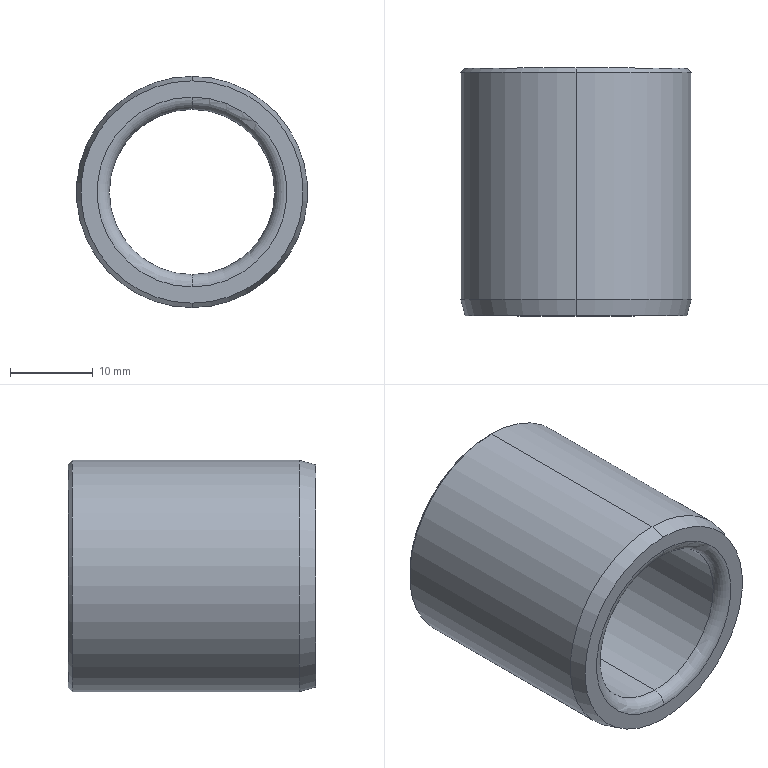Component | SolidWorks | BearingLiftingModule-1_CylinderLiftingModule-1_OFG01-d20-L30-1 | 1 solid | 14 faces | box 28 x 30 x 28 mm | volume 8928 mm3 | cone 4 | torus 4 | cylinder 4 | plane 2 | commonest cylinder face diameters 20 x2 28 x2
STEP:
#1=COLOUR_RGB('',0.7922,0.8196,0.9333);
#2=FILL_AREA_STYLE_COLOUR('',#1);
#3=FILL_AREA_STYLE('',(#2));
#4=SURFACE_STYLE_FILL_AREA(#3);
#5=SURFACE_SIDE_STYLE('',(#4));
#6=SURFACE_STYLE_USAGE(.BOTH.,#5);
#7=PRESENTATION_STYLE_ASSIGNMENT((#6));
#8=CARTESIAN_POINT('',(2.756,-1.622,1.711));
#9=VERTEX_POINT('',#8);
#10=CARTESIAN_POINT('',(2.756,-1.622,0.651));
#11=VERTEX_POINT('',#10);
#12=CARTESIAN_POINT('',(2.756,-1.622,1.181));
#13=DIRECTION('',(0.,-1.,0.));
#14=DIRECTION('',(0.,0.,1.));
#15=AXIS2_PLACEMENT_3D('',#12,#13,#14);
#16=CIRCLE('',#15,0.5301);
#17=EDGE_CURVE('',#9,#11,#16,.T.);
#18=ORIENTED_EDGE('',*,*,#17,.F.);
#19=CARTESIAN_POINT('',(2.756,-1.543,1.732));
#20=VERTEX_POINT('',#19);
#21=CARTESIAN_POINT('',(2.756,-1.622,1.711));
#22=DIRECTION('',(-0.,0.9659,0.2588));
#23=VECTOR('',#22,39.37);
#24=LINE('',#21,#23);
#25=EDGE_CURVE('',#9,#20,#24,.T.);
#26=ORIENTED_EDGE('',*,*,#25,.T.);
#27=CARTESIAN_POINT('',(2.756,-1.543,0.6299));
#28=VERTEX_POINT('',#27);
#29=CARTESIAN_POINT('',(2.756,-1.543,1.181));
#30=DIRECTION('',(0.,-1.,0.));
#31=DIRECTION('',(0.,0.,1.));
#32=AXIS2_PLACEMENT_3D('',#29,#30,#31);
#33=CIRCLE('',#32,0.5512);
#34=EDGE_CURVE('',#20,#28,#33,.T.);
#35=ORIENTED_EDGE('',*,*,#34,.T.);
#36=CARTESIAN_POINT('',(2.756,-1.622,0.651));
#37=DIRECTION('',(-0.,0.9659,-0.2588));
#38=VECTOR('',#37,39.37);
#39=LINE('',#36,#38);
#40=EDGE_CURVE('',#11,#28,#39,.T.);
#41=ORIENTED_EDGE('',*,*,#40,.F.);
#42=EDGE_LOOP('',(#18,#26,#35,#41));
#43=FACE_OUTER_BOUND('',#42,.T.);
#44=CARTESIAN_POINT('',(2.756,-1.622,1.181));
#45=DIRECTION('',(0.,1.,-0.));
#46=DIRECTION('',(0.,0.,-1.));
#47=AXIS2_PLACEMENT_3D('',#44,#45,#46);
#48=CONICAL_SURFACE('',#47,0.5301,0.2618);
#49=ADVANCED_FACE('',(#43),#48,.T.);
#50=CARTESIAN_POINT('',(2.756,-1.622,1.634));
#51=VERTEX_POINT('',#50);
#52=CARTESIAN_POINT('',(2.756,-1.622,0.7283));
#53=VERTEX_POINT('',#52);
#54=CARTESIAN_POINT('',(2.756,-1.622,1.181));
#55=DIRECTION('',(0.,-1.,0.));
#56=DIRECTION('',(0.,0.,1.));
#57=AXIS2_PLACEMENT_3D('',#54,#55,#56);
#58=CIRCLE('',#57,0.4528);
#59=EDGE_CURVE('',#51,#53,#58,.T.);
#60=ORIENTED_EDGE('',*,*,#59,.T.);
#61=CARTESIAN_POINT('',(2.756,-1.563,0.7874));
#62=VERTEX_POINT('',#61);
#63=CARTESIAN_POINT('',(2.756,-1.563,0.7283));
#64=DIRECTION('',(-1.,0.,0.));
#65=DIRECTION('',(0.,0.,1.));
#66=AXIS2_PLACEMENT_3D('',#63,#64,#65);
#67=CIRCLE('',#66,0.05906);
#68=EDGE_CURVE('',#53,#62,#67,.T.);
#69=ORIENTED_EDGE('',*,*,#68,.T.);
#70=CARTESIAN_POINT('',(2.756,-1.563,1.575));
#71=VERTEX_POINT('',#70);
#72=CARTESIAN_POINT('',(2.756,-1.563,1.181));
#73=DIRECTION('',(0.,-1.,0.));
#74=DIRECTION('',(0.,0.,1.));
#75=AXIS2_PLACEMENT_3D('',#72,#73,#74);
#76=CIRCLE('',#75,0.3937);
#77=EDGE_CURVE('',#71,#62,#76,.T.);
#78=ORIENTED_EDGE('',*,*,#77,.F.);
#79=CARTESIAN_POINT('',(2.756,-1.563,1.634));
#80=DIRECTION('',(1.,-0.,-0.));
#81=DIRECTION('',(0.,0.,-1.));
#82=AXIS2_PLACEMENT_3D('',#79,#80,#81);
#83=CIRCLE('',#82,0.05906);
#84=EDGE_CURVE('',#51,#71,#83,.T.);
#85=ORIENTED_EDGE('',*,*,#84,.F.);
#86=EDGE_LOOP('',(#60,#69,#78,#85));
#87=FACE_OUTER_BOUND('',#86,.T.);
#88=CARTESIAN_POINT('',(2.756,-1.563,1.181));
#89=DIRECTION('',(0.,-1.,0.));
#90=DIRECTION('',(0.,0.,1.));
#91=AXIS2_PLACEMENT_3D('',#88,#89,#90);
#92=TOROIDAL_SURFACE('',#91,0.4528,0.05906);
#93=ADVANCED_FACE('',(#87),#92,.T.);
#94=ORIENTED_EDGE('',*,*,#77,.T.);
#95=CARTESIAN_POINT('',(2.756,-0.5,0.7874));
#96=VERTEX_POINT('',#95);
#97=CARTESIAN_POINT('',(2.756,-1.622,0.7874));
#98=DIRECTION('',(0.,1.,-0.));
#99=VECTOR('',#98,39.37);
#100=LINE('',#97,#99);
#101=EDGE_CURVE('',#62,#96,#100,.T.);
#102=ORIENTED_EDGE('',*,*,#101,.T.);
#103=CARTESIAN_POINT('',(2.756,-0.5,1.575));
#104=VERTEX_POINT('',#103);
#105=CARTESIAN_POINT('',(2.756,-0.5,1.181));
#106=DIRECTION('',(0.,-1.,0.));
#107=DIRECTION('',(0.,0.,1.));
#108=AXIS2_PLACEMENT_3D('',#105,#106,#107);
#109=CIRCLE('',#108,0.3937);
#110=EDGE_CURVE('',#104,#96,#109,.T.);
#111=ORIENTED_EDGE('',*,*,#110,.F.);
#112=CARTESIAN_POINT('',(2.756,-1.622,1.575));
#113=DIRECTION('',(0.,1.,-0.));
#114=VECTOR('',#113,39.37);
#115=LINE('',#112,#114);
#116=EDGE_CURVE('',#71,#104,#115,.T.);
#117=ORIENTED_EDGE('',*,*,#116,.F.);
#118=EDGE_LOOP('',(#94,#102,#111,#117));
#119=FACE_OUTER_BOUND('',#118,.T.);
#120=CARTESIAN_POINT('',(2.756,-1.622,1.181));
#121=DIRECTION('',(0.,1.,-0.));
#122=DIRECTION('',(0.,0.,1.));
#123=AXIS2_PLACEMENT_3D('',#120,#121,#122);
#124=CYLINDRICAL_SURFACE('',#123,0.3937);
#125=ADVANCED_FACE('',(#119),#124,.F.);
#126=ORIENTED_EDGE('',*,*,#110,.T.);
#127=CARTESIAN_POINT('',(2.756,-0.4409,0.7283));
#128=VERTEX_POINT('',#127);
#129=CARTESIAN_POINT('',(2.756,-0.5,0.7283));
#130=DIRECTION('',(-1.,0.,0.));
#131=DIRECTION('',(0.,0.,1.));
#132=AXIS2_PLACEMENT_3D('',#129,#130,#131);
#133=CIRCLE('',#132,0.05906);
#134=EDGE_CURVE('',#96,#128,#133,.T.);
#135=ORIENTED_EDGE('',*,*,#134,.T.);
#136=CARTESIAN_POINT('',(2.756,-0.4409,1.634));
#137=VERTEX_POINT('',#136);
#138=CARTESIAN_POINT('',(2.756,-0.4409,1.181));
#139=DIRECTION('',(0.,-1.,0.));
#140=DIRECTION('',(0.,0.,1.));
#141=AXIS2_PLACEMENT_3D('',#138,#139,#140);
#142=CIRCLE('',#141,0.4528);
#143=EDGE_CURVE('',#137,#128,#142,.T.);
#144=ORIENTED_EDGE('',*,*,#143,.F.);
#145=CARTESIAN_POINT('',(2.756,-0.5,1.634));
#146=DIRECTION('',(1.,-0.,-0.));
#147=DIRECTION('',(0.,0.,-1.));
#148=AXIS2_PLACEMENT_3D('',#145,#146,#147);
#149=CIRCLE('',#148,0.05906);
#150=EDGE_CURVE('',#104,#137,#149,.T.);
#151=ORIENTED_EDGE('',*,*,#150,.F.);
#152=EDGE_LOOP('',(#126,#135,#144,#151));
#153=FACE_OUTER_BOUND('',#152,.T.);
#154=CARTESIAN_POINT('',(2.756,-0.5,1.181));
#155=DIRECTION('',(0.,-1.,0.));
#156=DIRECTION('',(0.,0.,1.));
#157=AXIS2_PLACEMENT_3D('',#154,#155,#156);
#158=TOROIDAL_SURFACE('',#157,0.4528,0.05906);
#159=ADVANCED_FACE('',(#153),#158,.T.);
#160=CARTESIAN_POINT('',(2.756,-1.543,1.181));
#161=DIRECTION('',(0.,-1.,0.));
#162=DIRECTION('',(0.,0.,1.));
#163=AXIS2_PLACEMENT_3D('',#160,#161,#162);
#164=CIRCLE('',#163,0.5512);
#165=EDGE_CURVE('',#28,#20,#164,.T.);
#166=ORIENTED_EDGE('',*,*,#165,.F.);
#167=CARTESIAN_POINT('',(2.756,-0.4606,0.6299));
#168=VERTEX_POINT('',#167);
#169=CARTESIAN_POINT('',(2.756,-1.622,0.6299));
#170=DIRECTION('',(0.,1.,-0.));
#171=VECTOR('',#170,39.37);
#172=LINE('',#169,#171);
#173=EDGE_CURVE('',#28,#168,#172,.T.);
#174=ORIENTED_EDGE('',*,*,#173,.T.);
#175=CARTESIAN_POINT('',(2.756,-0.4606,1.732));
#176=VERTEX_POINT('',#175);
#177=CARTESIAN_POINT('',(2.756,-0.4606,1.181));
#178=DIRECTION('',(0.,-1.,0.));
#179=DIRECTION('',(0.,0.,1.));
#180=AXIS2_PLACEMENT_3D('',#177,#178,#179);
#181=CIRCLE('',#180,0.5512);
#182=EDGE_CURVE('',#168,#176,#181,.T.);
#183=ORIENTED_EDGE('',*,*,#182,.T.);
#184=CARTESIAN_POINT('',(2.756,-1.622,1.732));
#185=DIRECTION('',(0.,1.,-0.));
#186=VECTOR('',#185,39.37);
#187=LINE('',#184,#186);
#188=EDGE_CURVE('',#20,#176,#187,.T.);
#189=ORIENTED_EDGE('',*,*,#188,.F.);
#190=EDGE_LOOP('',(#166,#174,#183,#189));
#191=FACE_OUTER_BOUND('',#190,.T.);
#192=CARTESIAN_POINT('',(2.756,-1.622,1.181));
#193=DIRECTION('',(0.,1.,-0.));
#194=DIRECTION('',(0.,0.,1.));
#195=AXIS2_PLACEMENT_3D('',#192,#193,#194);
#196=CYLINDRICAL_SURFACE('',#195,0.5512);
#197=ADVANCED_FACE('',(#191),#196,.T.);
#198=CARTESIAN_POINT('',(2.756,-0.4409,1.713));
#199=VERTEX_POINT('',#198);
#200=CARTESIAN_POINT('',(2.756,-0.4409,0.6496));
#201=VERTEX_POINT('',#200);
#202=CARTESIAN_POINT('',(2.756,-0.4409,1.181));
#203=DIRECTION('',(0.,-1.,0.));
#204=DIRECTION('',(0.,0.,1.));
#205=AXIS2_PLACEMENT_3D('',#202,#203,#204);
#206=CIRCLE('',#205,0.5315);
#207=EDGE_CURVE('',#199,#201,#206,.T.);
#208=ORIENTED_EDGE('',*,*,#207,.T.);
#209=CARTESIAN_POINT('',(2.756,-0.4606,0.6299));
#210=DIRECTION('',(-0.,-0.7071,-0.7071));
#211=VECTOR('',#210,39.37);
#212=LINE('',#209,#211);
#213=EDGE_CURVE('',#201,#168,#212,.T.);
#214=ORIENTED_EDGE('',*,*,#213,.T.);
#215=CARTESIAN_POINT('',(2.756,-0.4606,1.181));
#216=DIRECTION('',(0.,-1.,0.));
#217=DIRECTION('',(0.,0.,1.));
#218=AXIS2_PLACEMENT_3D('',#215,#216,#217);
#219=CIRCLE('',#218,0.5512);
#220=EDGE_CURVE('',#176,#168,#219,.T.);
#221=ORIENTED_EDGE('',*,*,#220,.F.);
#222=CARTESIAN_POINT('',(2.756,-0.4606,1.732));
#223=DIRECTION('',(0.,-0.7071,0.7071));
#224=VECTOR('',#223,39.37);
#225=LINE('',#222,#224);
#226=EDGE_CURVE('',#199,#176,#225,.T.);
#227=ORIENTED_EDGE('',*,*,#226,.F.);
#228=EDGE_LOOP('',(#208,#214,#221,#227));
#229=FACE_OUTER_BOUND('',#228,.T.);
#230=CARTESIAN_POINT('',(2.756,-0.4606,1.181));
#231=DIRECTION('',(0.,-1.,0.));
#232=DIRECTION('',(0.,0.,1.));
#233=AXIS2_PLACEMENT_3D('',#230,#231,#232);
#234=CONICAL_SURFACE('',#233,0.5512,0.7854);
#235=ADVANCED_FACE('',(#229),#234,.T.);
#236=ORIENTED_EDGE('',*,*,#213,.F.);
#237=CARTESIAN_POINT('',(2.756,-0.4409,1.181));
#238=DIRECTION('',(0.,-1.,0.));
#239=DIRECTION('',(0.,0.,1.));
#240=AXIS2_PLACEMENT_3D('',#237,#238,#239);
#241=CIRCLE('',#240,0.5315);
#242=EDGE_CURVE('',#201,#199,#241,.T.);
#243=ORIENTED_EDGE('',*,*,#242,.T.);
#244=ORIENTED_EDGE('',*,*,#226,.T.);
#245=ORIENTED_EDGE('',*,*,#182,.F.);
#246=EDGE_LOOP('',(#236,#243,#244,#245));
#247=FACE_OUTER_BOUND('',#246,.T.);
#248=CARTESIAN_POINT('',(2.756,-0.4606,1.181));
#249=DIRECTION('',(0.,-1.,0.));
#250=DIRECTION('',(0.,0.,1.));
#251=AXIS2_PLACEMENT_3D('',#248,#249,#250);
#252=CONICAL_SURFACE('',#251,0.5512,0.7854);
#253=ADVANCED_FACE('',(#247),#252,.T.);
#254=ORIENTED_EDGE('',*,*,#173,.F.);
#255=ORIENTED_EDGE('',*,*,#34,.F.);
#256=ORIENTED_EDGE('',*,*,#188,.T.);
#257=ORIENTED_EDGE('',*,*,#220,.T.);
#258=EDGE_LOOP('',(#254,#255,#256,#257));
#259=FACE_OUTER_BOUND('',#258,.T.);
#260=CARTESIAN_POINT('',(2.756,-1.622,1.181));
#261=DIRECTION('',(0.,1.,-0.));
#262=DIRECTION('',(0.,0.,1.));
#263=AXIS2_PLACEMENT_3D('',#260,#261,#262);
#264=CYLINDRICAL_SURFACE('',#263,0.5512);
#265=ADVANCED_FACE('',(#259),#264,.T.);
#266=ORIENTED_EDGE('',*,*,#207,.F.);
#267=ORIENTED_EDGE('',*,*,#242,.F.);
#268=EDGE_LOOP('',(#266,#267));
#269=FACE_OUTER_BOUND('',#268,.T.);
#270=ORIENTED_EDGE('',*,*,#143,.T.);
#271=CARTESIAN_POINT('',(2.756,-0.4409,1.181));
#272=DIRECTION('',(0.,-1.,0.));
#273=DIRECTION('',(0.,0.,1.));
#274=AXIS2_PLACEMENT_3D('',#271,#272,#273);
#275=CIRCLE('',#274,0.4528);
#276=EDGE_CURVE('',#128,#137,#275,.T.);
#277=ORIENTED_EDGE('',*,*,#276,.T.);
#278=EDGE_LOOP('',(#270,#277));
#279=FACE_BOUND('',#278,.T.);
#280=CARTESIAN_POINT('',(2.224,-0.4409,1.181));
#281=DIRECTION('',(0.,1.,-0.));
#282=DIRECTION('',(-0.,-0.,-1.));
#283=AXIS2_PLACEMENT_3D('',#280,#281,#282);
#284=PLANE('',#283);
#285=ADVANCED_FACE('',(#269,#279),#284,.T.);
#286=ORIENTED_EDGE('',*,*,#134,.F.);
#287=CARTESIAN_POINT('',(2.756,-0.5,1.181));
#288=DIRECTION('',(0.,-1.,0.));
#289=DIRECTION('',(0.,0.,1.));
#290=AXIS2_PLACEMENT_3D('',#287,#288,#289);
#291=CIRCLE('',#290,0.3937);
#292=EDGE_CURVE('',#96,#104,#291,.T.);
#293=ORIENTED_EDGE('',*,*,#292,.T.);
#294=ORIENTED_EDGE('',*,*,#150,.T.);
#295=ORIENTED_EDGE('',*,*,#276,.F.);
#296=EDGE_LOOP('',(#286,#293,#294,#295));
#297=FACE_OUTER_BOUND('',#296,.T.);
#298=CARTESIAN_POINT('',(2.756,-0.5,1.181));
#299=DIRECTION('',(0.,-1.,0.));
#300=DIRECTION('',(0.,0.,1.));
#301=AXIS2_PLACEMENT_3D('',#298,#299,#300);
#302=TOROIDAL_SURFACE('',#301,0.4528,0.05906);
#303=ADVANCED_FACE('',(#297),#302,.T.);
#304=ORIENTED_EDGE('',*,*,#101,.F.);
#305=CARTESIAN_POINT('',(2.756,-1.563,1.181));
#306=DIRECTION('',(0.,-1.,0.));
#307=DIRECTION('',(0.,0.,1.));
#308=AXIS2_PLACEMENT_3D('',#305,#306,#307);
#309=CIRCLE('',#308,0.3937);
#310=EDGE_CURVE('',#62,#71,#309,.T.);
#311=ORIENTED_EDGE('',*,*,#310,.T.);
#312=ORIENTED_EDGE('',*,*,#116,.T.);
#313=ORIENTED_EDGE('',*,*,#292,.F.);
#314=EDGE_LOOP('',(#304,#311,#312,#313));
#315=FACE_OUTER_BOUND('',#314,.T.);
#316=CARTESIAN_POINT('',(2.756,-1.622,1.181));
#317=DIRECTION('',(0.,1.,-0.));
#318=DIRECTION('',(0.,0.,1.));
#319=AXIS2_PLACEMENT_3D('',#316,#317,#318);
#320=CYLINDRICAL_SURFACE('',#319,0.3937);
#321=ADVANCED_FACE('',(#315),#320,.F.);
#322=ORIENTED_EDGE('',*,*,#68,.F.);
#323=CARTESIAN_POINT('',(2.756,-1.622,1.181));
#324=DIRECTION('',(0.,-1.,0.));
#325=DIRECTION('',(0.,0.,1.));
#326=AXIS2_PLACEMENT_3D('',#323,#324,#325);
#327=CIRCLE('',#326,0.4528);
#328=EDGE_CURVE('',#53,#51,#327,.T.);
#329=ORIENTED_EDGE('',*,*,#328,.T.);
#330=ORIENTED_EDGE('',*,*,#84,.T.);
#331=ORIENTED_EDGE('',*,*,#310,.F.);
#332=EDGE_LOOP('',(#322,#329,#330,#331));
#333=FACE_OUTER_BOUND('',#332,.T.);
#334=CARTESIAN_POINT('',(2.756,-1.563,1.181));
#335=DIRECTION('',(0.,-1.,0.));
#336=DIRECTION('',(0.,0.,1.));
#337=AXIS2_PLACEMENT_3D('',#334,#335,#336);
#338=TOROIDAL_SURFACE('',#337,0.4528,0.05906);
#339=ADVANCED_FACE('',(#333),#338,.T.);
#340=CARTESIAN_POINT('',(2.756,-1.622,1.181));
#341=DIRECTION('',(0.,-1.,0.));
#342=DIRECTION('',(0.,0.,1.));
#343=AXIS2_PLACEMENT_3D('',#340,#341,#342);
#344=CIRCLE('',#343,0.5301);
#345=EDGE_CURVE('',#11,#9,#344,.T.);
#346=ORIENTED_EDGE('',*,*,#345,.T.);
#347=ORIENTED_EDGE('',*,*,#17,.T.);
#348=EDGE_LOOP('',(#346,#347));
#349=FACE_OUTER_BOUND('',#348,.T.);
#350=ORIENTED_EDGE('',*,*,#59,.F.);
#351=ORIENTED_EDGE('',*,*,#328,.F.);
#352=EDGE_LOOP('',(#350,#351));
#353=FACE_BOUND('',#352,.T.);
#354=CARTESIAN_POINT('',(2.303,-1.622,1.181));
#355=DIRECTION('',(0.,-1.,0.));
#356=DIRECTION('',(-1.,0.,0.));
#357=AXIS2_PLACEMENT_3D('',#354,#355,#356);
#358=PLANE('',#357);
#359=ADVANCED_FACE('',(#349,#353),#358,.T.);
#360=ORIENTED_EDGE('',*,*,#25,.F.);
#361=ORIENTED_EDGE('',*,*,#345,.F.);
#362=ORIENTED_EDGE('',*,*,#40,.T.);
#363=ORIENTED_EDGE('',*,*,#165,.T.);
#364=EDGE_LOOP('',(#360,#361,#362,#363));
#365=FACE_OUTER_BOUND('',#364,.T.);
#366=CARTESIAN_POINT('',(2.756,-1.622,1.181));
#367=DIRECTION('',(0.,1.,-0.));
#368=DIRECTION('',(0.,0.,-1.));
#369=AXIS2_PLACEMENT_3D('',#366,#367,#368);
#370=CONICAL_SURFACE('',#369,0.5301,0.2618);
#371=ADVANCED_FACE('',(#365),#370,.T.);
#372=CLOSED_SHELL('',(#49,#93,#125,#159,#197,#235,#253,#265,#285,#303,#321,#339,#359,#371));
#373=MANIFOLD_SOLID_BREP('',#372);
#374=STYLED_ITEM('',(#7),#373);
#375=PRESENTATION_LAYER_ASSIGNMENT('','',(#374));
#376=CARTESIAN_POINT('',(0.,0.,0.));
#377=DIRECTION('',(0.,0.,1.));
#378=DIRECTION('',(1.,0.,0.));
#379=AXIS2_PLACEMENT_3D('',#376,#377,#378);
#380=(LENGTH_UNIT()NAMED_UNIT(*)SI_UNIT($,.METRE.));
#381=LENGTH_MEASURE_WITH_UNIT(LENGTH_MEASURE(0.0254),#380);
#382=DIMENSIONAL_EXPONENTS(1.,0.,0.,0.,0.,0.,0.);
#383=(CONVERSION_BASED_UNIT('',#381)LENGTH_UNIT()NAMED_UNIT(#382));
#384=UNCERTAINTY_MEASURE_WITH_UNIT(LENGTH_MEASURE(0.00001),#383,'','');
#385=(NAMED_UNIT(*)PLANE_ANGLE_UNIT()SI_UNIT($,.RADIAN.));
#386=(NAMED_UNIT(*)SI_UNIT($,.STERADIAN.)SOLID_ANGLE_UNIT());
#387=(GEOMETRIC_REPRESENTATION_CONTEXT(3)GLOBAL_UNCERTAINTY_ASSIGNED_CONTEXT((#384))GLOBAL_UNIT_ASSIGNED_CONTEXT((#383,#385,#386))REPRESENTATION_CONTEXT('',''));
#388=ADVANCED_BREP_SHAPE_REPRESENTATION('',(#373,#379),#387);
#389=(LENGTH_UNIT()NAMED_UNIT(*)SI_UNIT($,.METRE.));
#390=LENGTH_MEASURE_WITH_UNIT(LENGTH_MEASURE(0.0254),#389);
#391=DIMENSIONAL_EXPONENTS(1.,0.,0.,0.,0.,0.,0.);
#392=(CONVERSION_BASED_UNIT('',#390)LENGTH_UNIT()NAMED_UNIT(#391));
#393=UNCERTAINTY_MEASURE_WITH_UNIT(LENGTH_MEASURE(0.00001),#392,'','');
#394=(NAMED_UNIT(*)PLANE_ANGLE_UNIT()SI_UNIT($,.RADIAN.));
#395=(NAMED_UNIT(*)SI_UNIT($,.STERADIAN.)SOLID_ANGLE_UNIT());
#396=(GEOMETRIC_REPRESENTATION_CONTEXT(3)GLOBAL_UNCERTAINTY_ASSIGNED_CONTEXT((#393))GLOBAL_UNIT_ASSIGNED_CONTEXT((#392,#394,#395))REPRESENTATION_CONTEXT('',''));
#397=MECHANICAL_DESIGN_GEOMETRIC_PRESENTATION_REPRESENTATION('',(#374),#396);